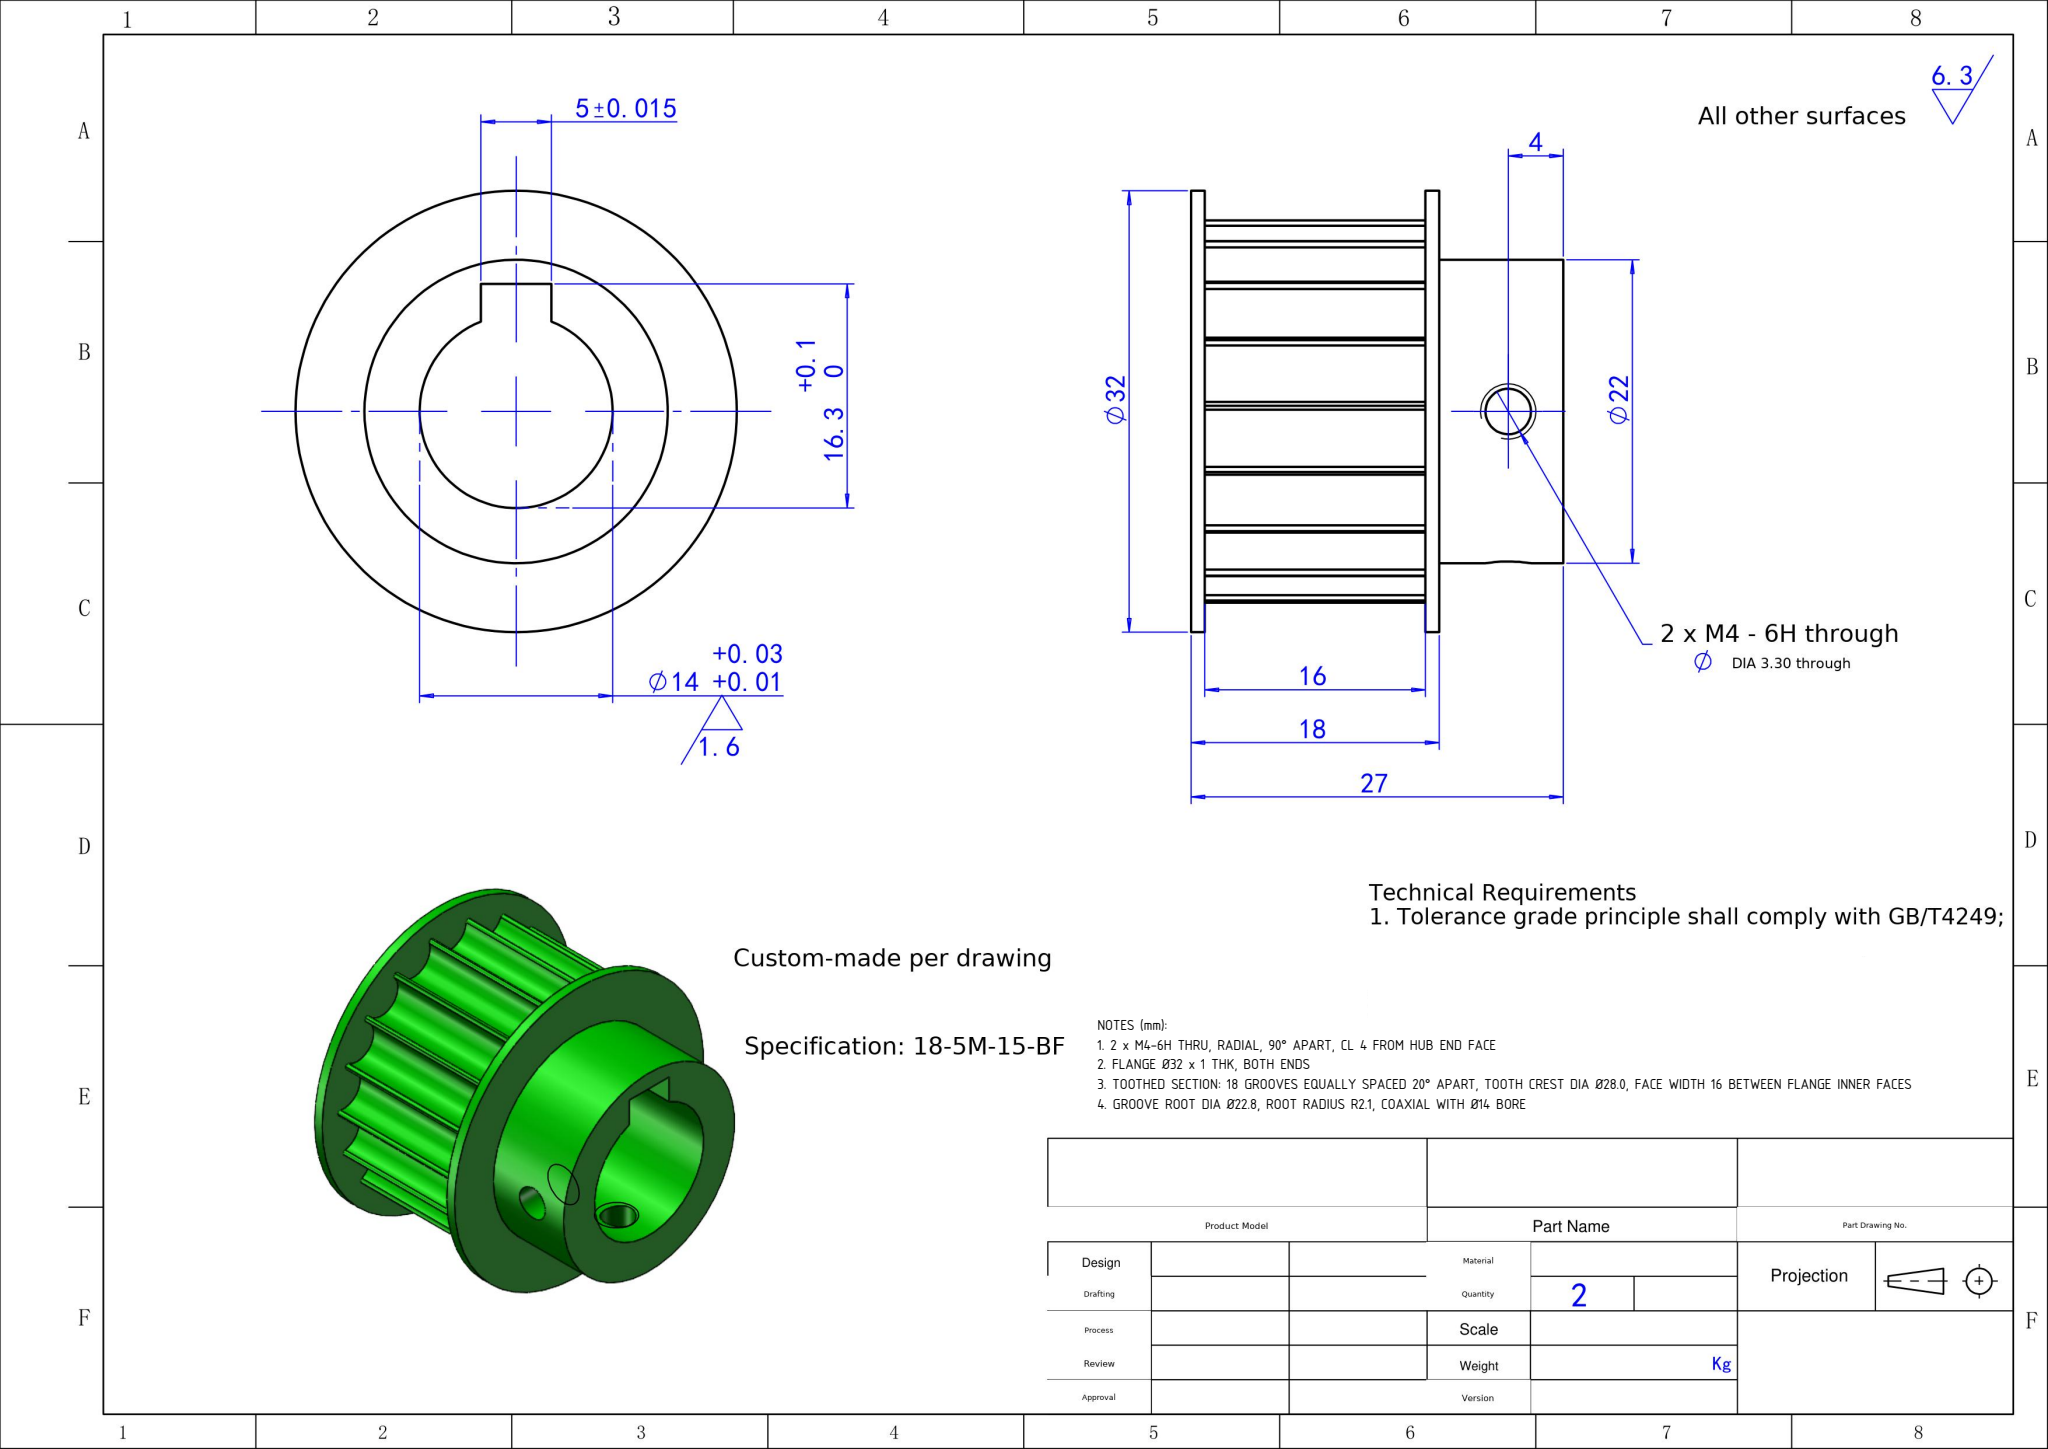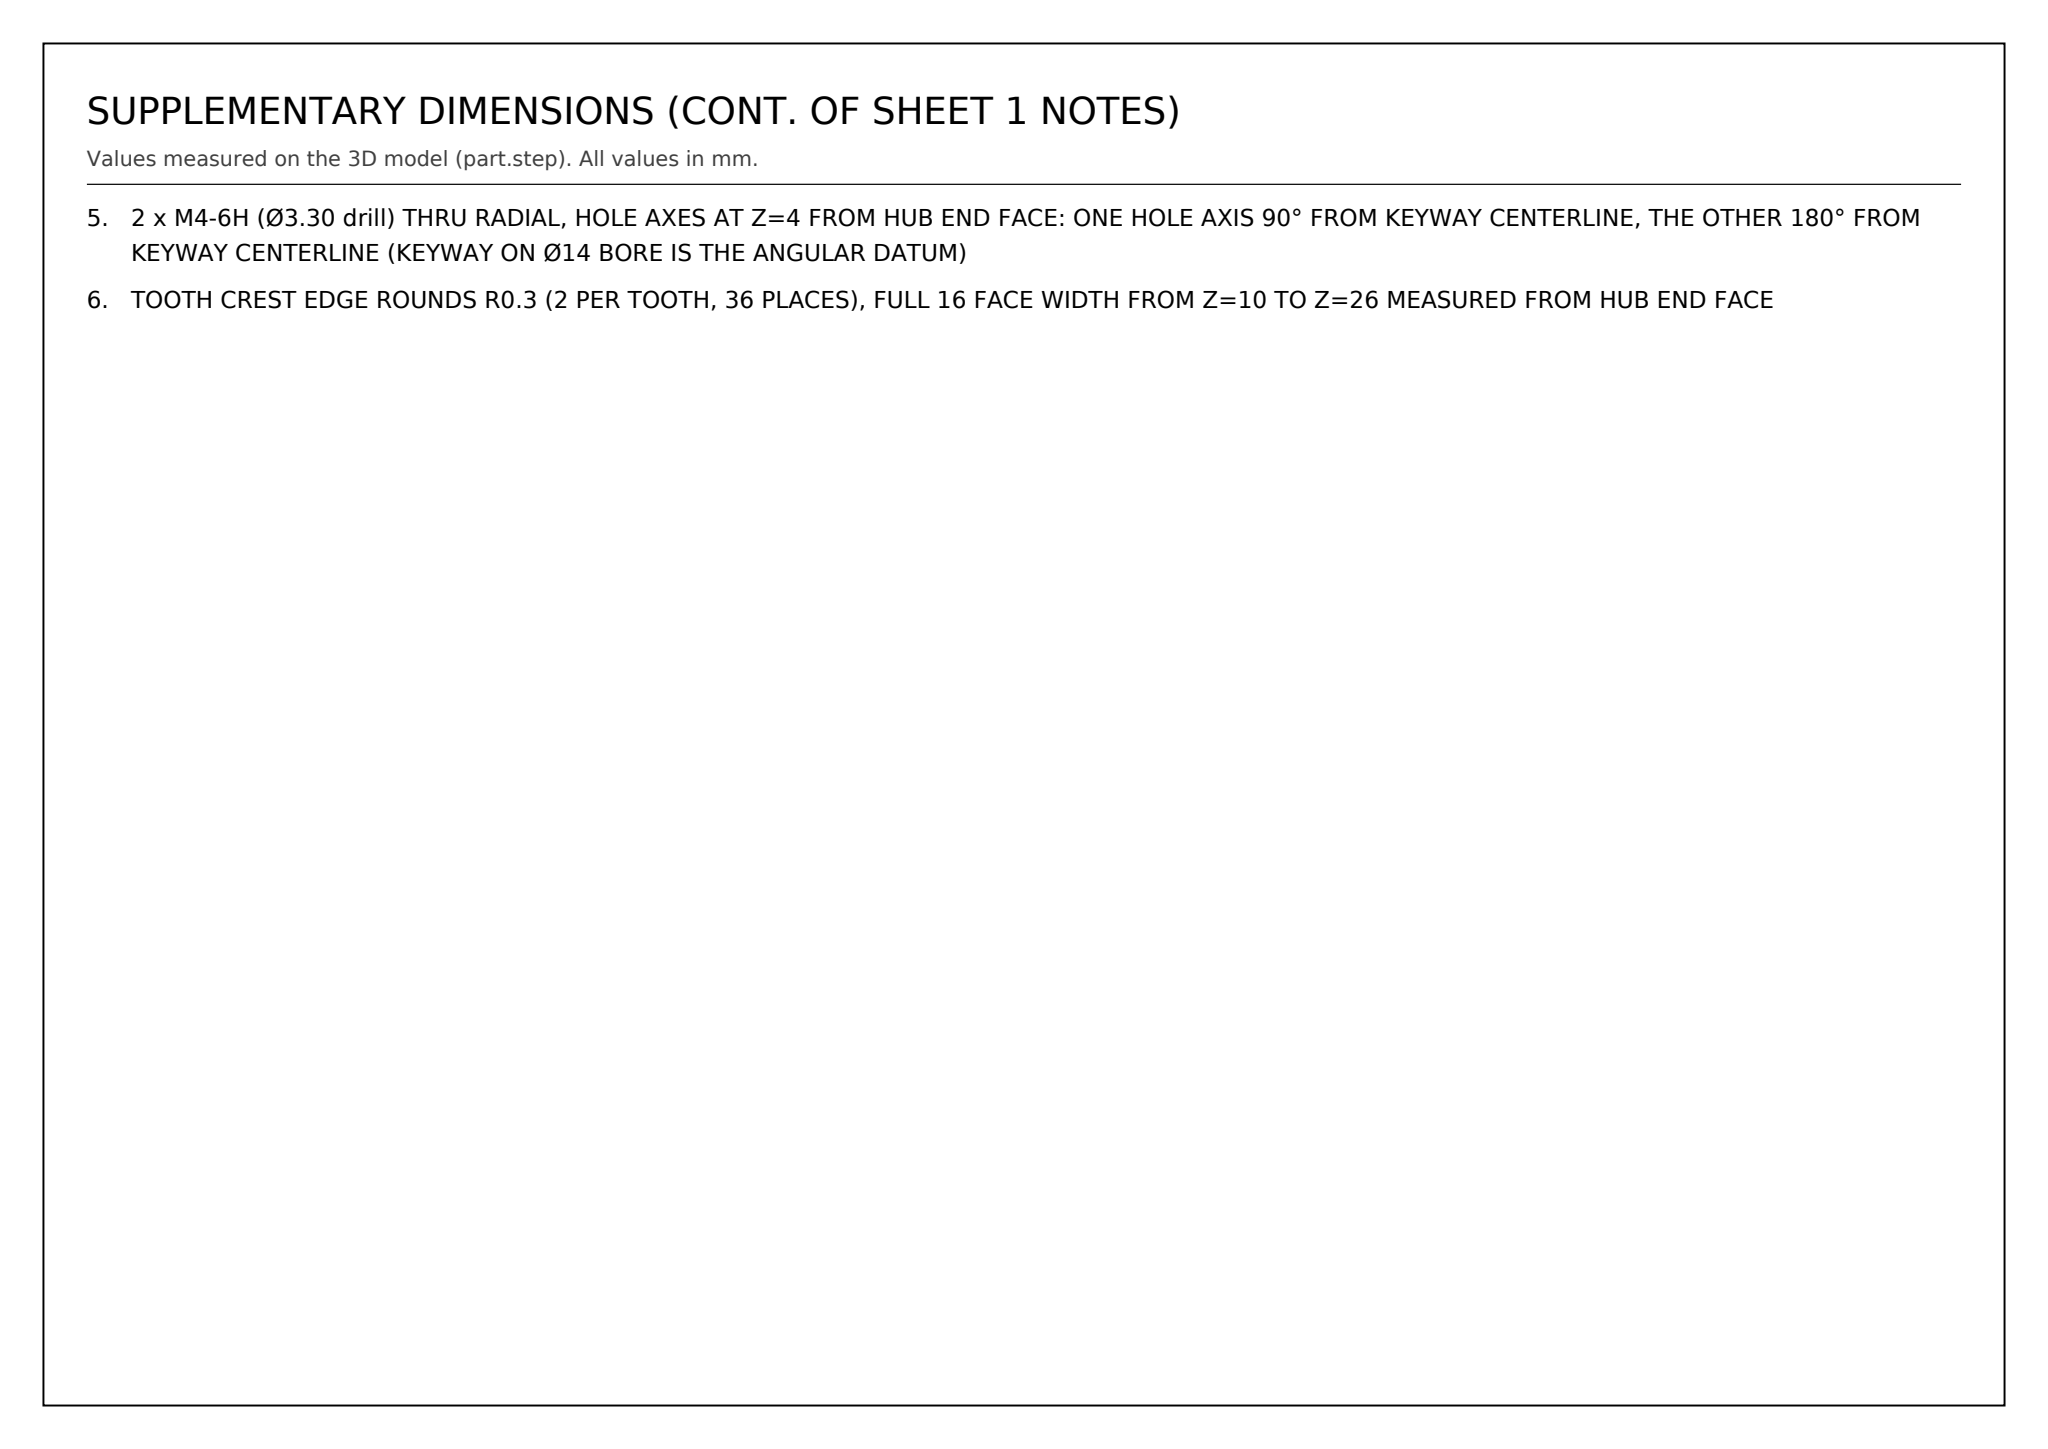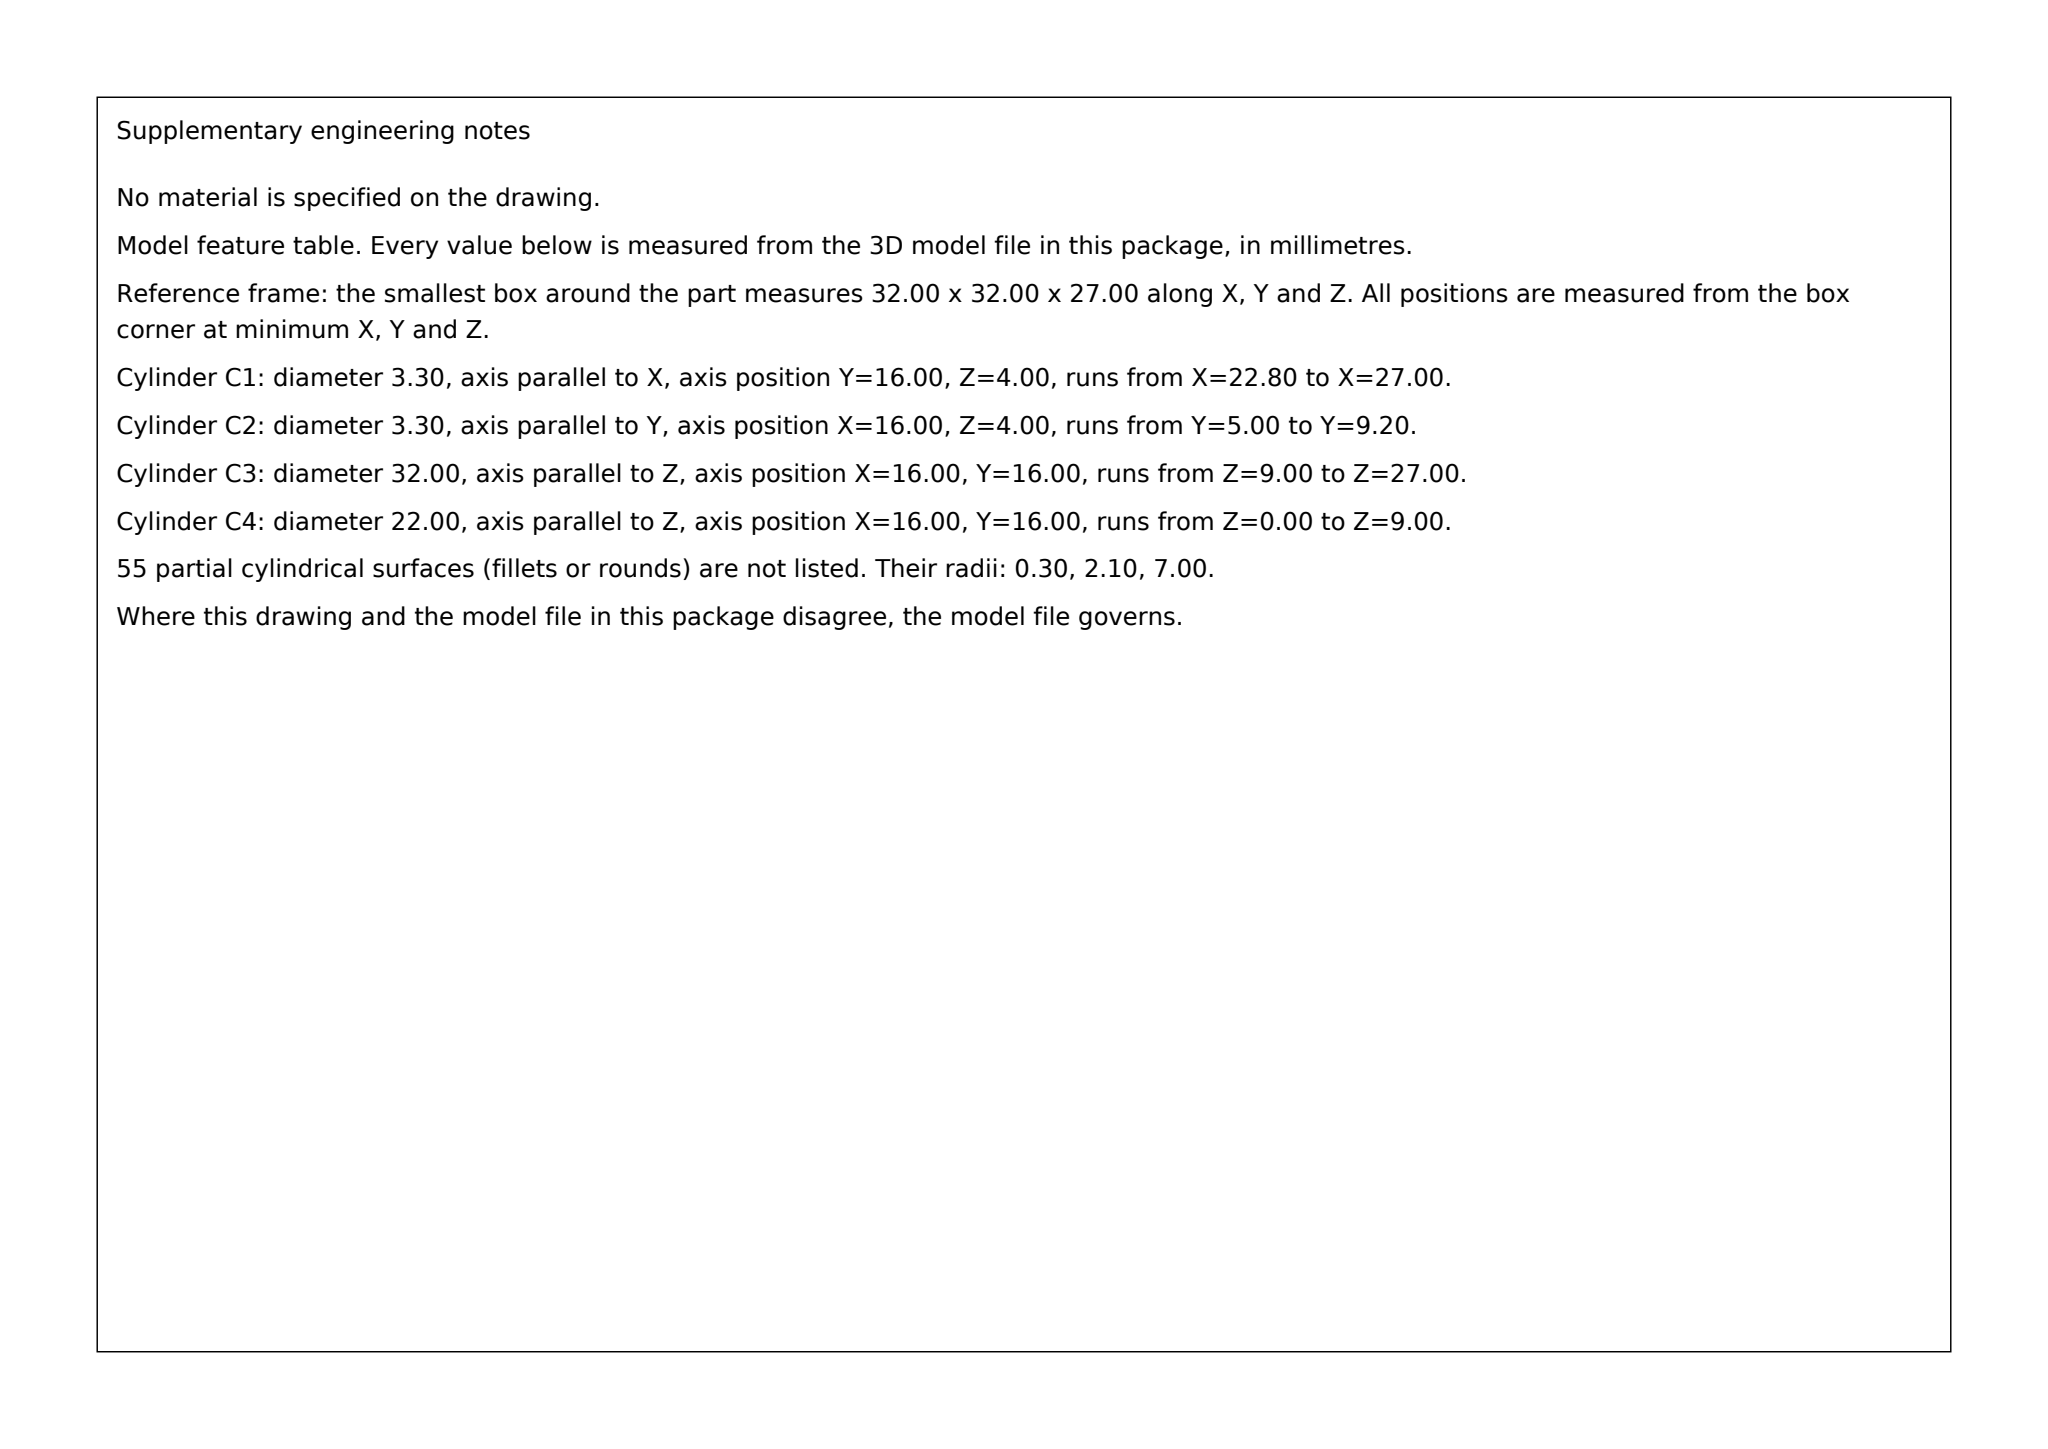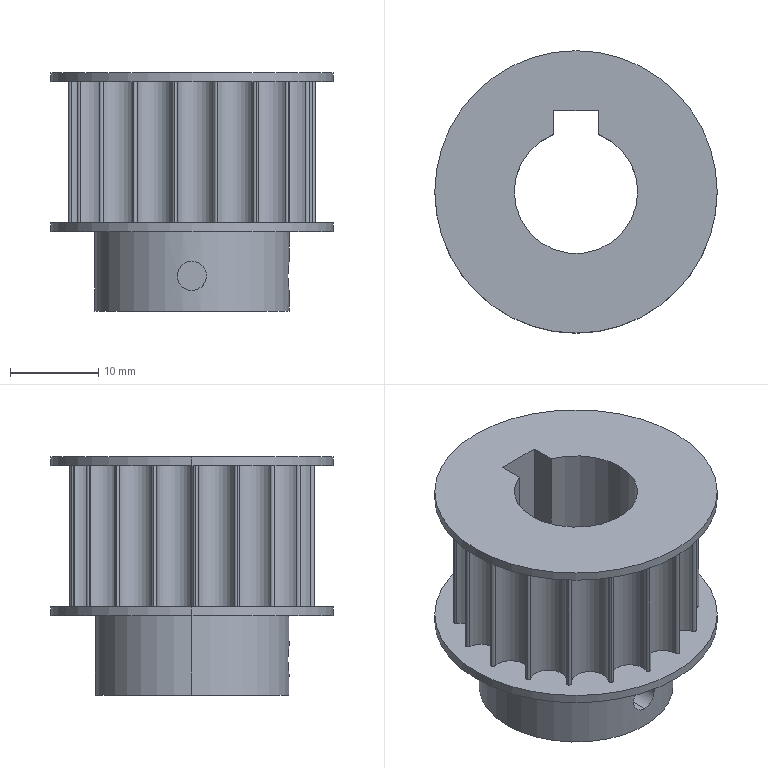Part | SolidWorks | mm | 1 solid | 93 faces | box 32 x 32 x 27 mm | volume 7780 mm3 | cylinder 85 | plane 8 | commonest cylinder face diameters 0.6 x45 4.2 x27 3.3 x4 32 x4 14 x3 22 x2
Drawing notes:
2 x M4-6H THRU, RADIAL, 90° APART, CL 4 FROM HUB END FACE | from the solid: Ø3.3 cyls: axis x at (y=16,z=4) and axis y at (x=16,z=4) -> two radial holes 90° apart, CL z=4
FLANGE Ø32 x 1 THK, BOTH ENDS | from the solid: Ø32 cylinders length 1 at each end; z planes at 0/1 and 26/27
TOOTHED SECTION: 18 GROOVES EQUALLY SPACED 20° APART, TOOTH CREST DIA Ø28.0, FACE WIDTH 16 BETWEEN FLANGE INNER FACES | from the solid: eighteen 4.2 dia z-cylinders L16.0 (groove roots) + 0.6 dia z-cylinders at R13.70 from axis (16,16) giving crest Ø28.0; z planes 10 and 26
GROOVE ROOT DIA Ø22.8, ROOT RADIUS R2.1, COAXIAL WITH Ø14 BORE | from the solid: 4.2 dia z-cylinders L16.0 at R13.51 from axis (16,16) -> root Ø22.8; 14.0 dia z-cylinder at (16,16) L27
2 x M4-6H (Ø3.30 drill) THRU RADIAL, HOLE AXES AT Z=4 FROM HUB END FACE: ONE HOLE AXIS 90° FROM KEYWAY CENTERLINE, THE OTHER 180° FROM KEYWAY CENTERLINE (KEYWAY ON Ø14 BORE IS THE ANGULAR DATUM) | from the solid: cylinders: hole/bore Ø3.3 axis x at [y=16, z=4] (+X side) and hole/bore Ø3.3 axis y at [x=16, z=4] (-Y side); keyway axis planes x=13.5 & x=18.6 with y=25.3 face (+Y side) on Ø14 bore centered at (16,16)
TOOTH CREST EDGE ROUNDS R0.3 (2 PER TOOTH, 36 PLACES), FULL 16 FACE WIDTH FROM Z=10 TO Z=26 MEASURED FROM HUB END FACE | from the solid: cylinders 'convex arc (round/outer radius)' dia 0.6 (= R0.3), axis z, from 10.0 to 26.0, 36 instances around tooth crests